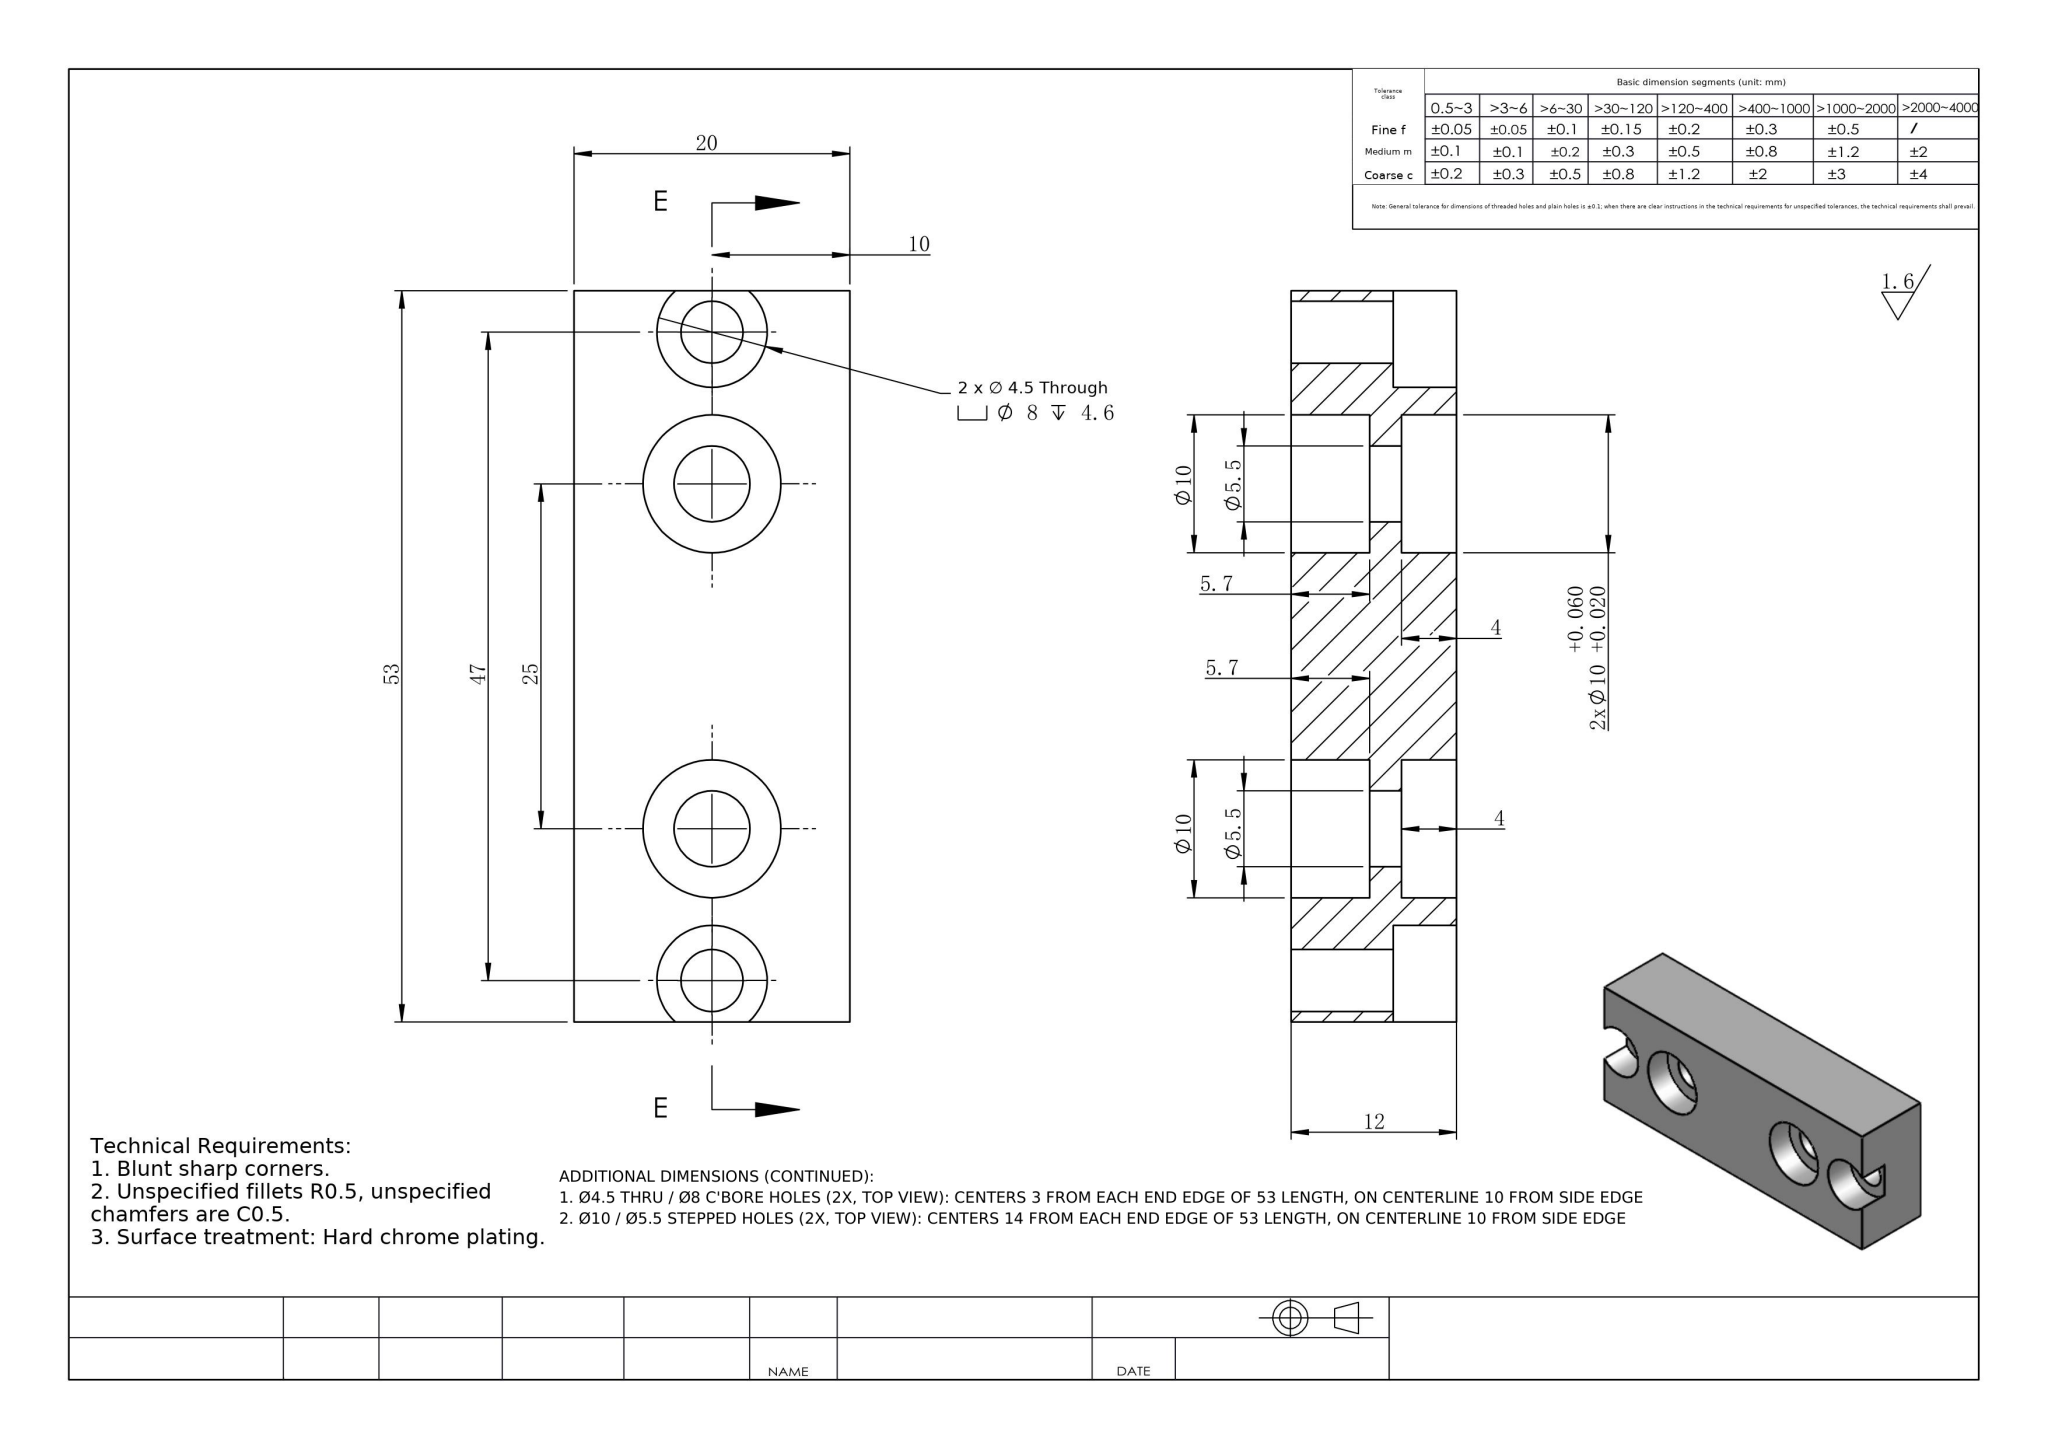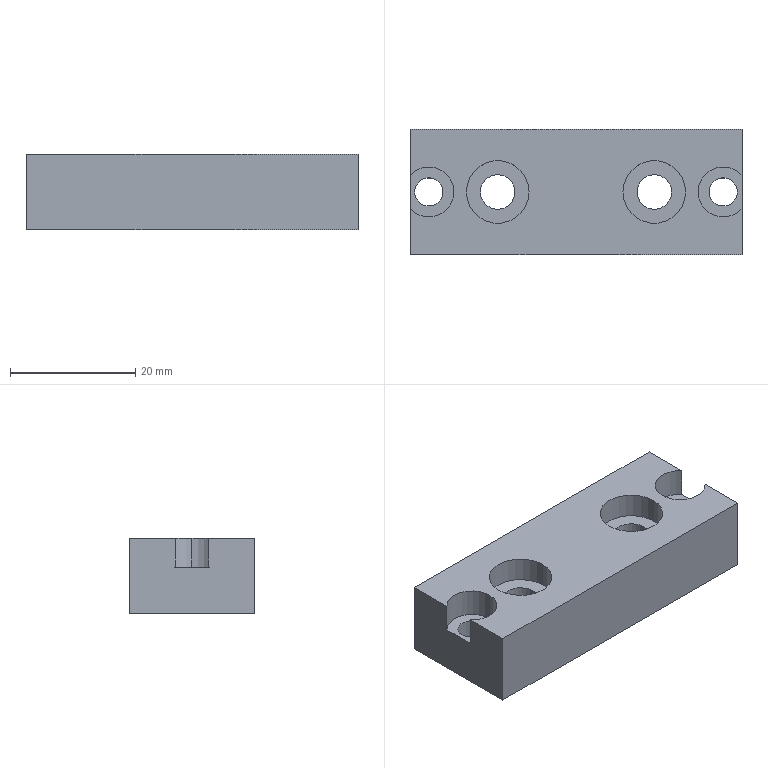Part | NX | mm | 1 solid | 31 faces | box 53 x 20 x 12 mm | volume 10423 mm3 | cylinder 19 | plane 12 | commonest cylinder face diameters 10 x8 5.5 x4 4.5 x4 8 x3
STEP:
#1=COLOUR_RGB('',1.,1.,1.);
#2=FILL_AREA_STYLE_COLOUR('',#1);
#3=FILL_AREA_STYLE('',(#2));
#4=SURFACE_STYLE_FILL_AREA(#3);
#5=SURFACE_SIDE_STYLE('',(#4));
#6=SURFACE_STYLE_USAGE(.BOTH.,#5);
#7=PRESENTATION_STYLE_ASSIGNMENT((#6));
#8=CARTESIAN_POINT('',(44.,-10.,5.7));
#9=VERTEX_POINT('',#8);
#10=CARTESIAN_POINT('',(34.,-10.,5.7));
#11=VERTEX_POINT('',#10);
#12=CARTESIAN_POINT('',(39.,-10.,5.7));
#13=DIRECTION('',(0.,0.,-1.));
#14=DIRECTION('',(-1.,0.,0.));
#15=AXIS2_PLACEMENT_3D('',#12,#13,#14);
#16=CIRCLE('',#15,5.);
#17=EDGE_CURVE('',#9,#11,#16,.T.);
#18=ORIENTED_EDGE('',*,*,#17,.F.);
#19=CARTESIAN_POINT('',(44.,-10.,0.));
#20=VERTEX_POINT('',#19);
#21=CARTESIAN_POINT('',(44.,-10.,0.));
#22=DIRECTION('',(0.,0.,-1.));
#23=VECTOR('',#22,1000.);
#24=LINE('',#21,#23);
#25=EDGE_CURVE('',#9,#20,#24,.T.);
#26=ORIENTED_EDGE('',*,*,#25,.T.);
#27=CARTESIAN_POINT('',(34.,-10.,0.));
#28=VERTEX_POINT('',#27);
#29=CARTESIAN_POINT('',(39.,-10.,0.));
#30=DIRECTION('',(0.,0.,-1.));
#31=DIRECTION('',(-1.,0.,0.));
#32=AXIS2_PLACEMENT_3D('',#29,#30,#31);
#33=CIRCLE('',#32,5.);
#34=EDGE_CURVE('',#20,#28,#33,.T.);
#35=ORIENTED_EDGE('',*,*,#34,.T.);
#36=CARTESIAN_POINT('',(34.,-10.,0.));
#37=DIRECTION('',(0.,0.,-1.));
#38=VECTOR('',#37,1000.);
#39=LINE('',#36,#38);
#40=EDGE_CURVE('',#11,#28,#39,.T.);
#41=ORIENTED_EDGE('',*,*,#40,.F.);
#42=EDGE_LOOP('',(#18,#26,#35,#41));
#43=FACE_OUTER_BOUND('',#42,.T.);
#44=CARTESIAN_POINT('',(39.,-10.,0.));
#45=DIRECTION('',(0.,0.,-1.));
#46=DIRECTION('',(-1.,0.,0.));
#47=AXIS2_PLACEMENT_3D('',#44,#45,#46);
#48=CYLINDRICAL_SURFACE('',#47,5.);
#49=ADVANCED_FACE('',(#43),#48,.F.);
#50=CARTESIAN_POINT('',(36.25,-10.,8.));
#51=VERTEX_POINT('',#50);
#52=CARTESIAN_POINT('',(41.75,-10.,8.));
#53=VERTEX_POINT('',#52);
#54=CARTESIAN_POINT('',(39.,-10.,8.));
#55=DIRECTION('',(0.,0.,1.));
#56=DIRECTION('',(1.,0.,0.));
#57=AXIS2_PLACEMENT_3D('',#54,#55,#56);
#58=CIRCLE('',#57,2.75);
#59=EDGE_CURVE('',#51,#53,#58,.T.);
#60=ORIENTED_EDGE('',*,*,#59,.T.);
#61=CARTESIAN_POINT('',(41.75,-10.,5.7));
#62=VERTEX_POINT('',#61);
#63=CARTESIAN_POINT('',(41.75,-10.,0.));
#64=DIRECTION('',(0.,0.,-1.));
#65=VECTOR('',#64,1000.);
#66=LINE('',#63,#65);
#67=EDGE_CURVE('',#53,#62,#66,.T.);
#68=ORIENTED_EDGE('',*,*,#67,.T.);
#69=CARTESIAN_POINT('',(36.25,-10.,5.7));
#70=VERTEX_POINT('',#69);
#71=CARTESIAN_POINT('',(39.,-10.,5.7));
#72=DIRECTION('',(0.,0.,-1.));
#73=DIRECTION('',(-1.,0.,0.));
#74=AXIS2_PLACEMENT_3D('',#71,#72,#73);
#75=CIRCLE('',#74,2.75);
#76=EDGE_CURVE('',#62,#70,#75,.T.);
#77=ORIENTED_EDGE('',*,*,#76,.T.);
#78=CARTESIAN_POINT('',(36.25,-10.,0.));
#79=DIRECTION('',(0.,0.,-1.));
#80=VECTOR('',#79,1000.);
#81=LINE('',#78,#80);
#82=EDGE_CURVE('',#51,#70,#81,.T.);
#83=ORIENTED_EDGE('',*,*,#82,.F.);
#84=EDGE_LOOP('',(#60,#68,#77,#83));
#85=FACE_OUTER_BOUND('',#84,.T.);
#86=CARTESIAN_POINT('',(39.,-10.,0.));
#87=DIRECTION('',(0.,0.,-1.));
#88=DIRECTION('',(-1.,0.,0.));
#89=AXIS2_PLACEMENT_3D('',#86,#87,#88);
#90=CYLINDRICAL_SURFACE('',#89,2.75);
#91=ADVANCED_FACE('',(#85),#90,.F.);
#92=CARTESIAN_POINT('',(19.,-10.,5.7));
#93=VERTEX_POINT('',#92);
#94=CARTESIAN_POINT('',(9.,-10.,5.7));
#95=VERTEX_POINT('',#94);
#96=CARTESIAN_POINT('',(14.,-10.,5.7));
#97=DIRECTION('',(0.,0.,-1.));
#98=DIRECTION('',(-1.,0.,0.));
#99=AXIS2_PLACEMENT_3D('',#96,#97,#98);
#100=CIRCLE('',#99,5.);
#101=EDGE_CURVE('',#93,#95,#100,.T.);
#102=ORIENTED_EDGE('',*,*,#101,.F.);
#103=CARTESIAN_POINT('',(19.,-10.,0.));
#104=VERTEX_POINT('',#103);
#105=CARTESIAN_POINT('',(19.,-10.,0.));
#106=DIRECTION('',(0.,0.,-1.));
#107=VECTOR('',#106,1000.);
#108=LINE('',#105,#107);
#109=EDGE_CURVE('',#93,#104,#108,.T.);
#110=ORIENTED_EDGE('',*,*,#109,.T.);
#111=CARTESIAN_POINT('',(9.,-10.,0.));
#112=VERTEX_POINT('',#111);
#113=CARTESIAN_POINT('',(14.,-10.,0.));
#114=DIRECTION('',(0.,0.,-1.));
#115=DIRECTION('',(-1.,0.,0.));
#116=AXIS2_PLACEMENT_3D('',#113,#114,#115);
#117=CIRCLE('',#116,5.);
#118=EDGE_CURVE('',#104,#112,#117,.T.);
#119=ORIENTED_EDGE('',*,*,#118,.T.);
#120=CARTESIAN_POINT('',(9.,-10.,0.));
#121=DIRECTION('',(0.,0.,-1.));
#122=VECTOR('',#121,1000.);
#123=LINE('',#120,#122);
#124=EDGE_CURVE('',#95,#112,#123,.T.);
#125=ORIENTED_EDGE('',*,*,#124,.F.);
#126=EDGE_LOOP('',(#102,#110,#119,#125));
#127=FACE_OUTER_BOUND('',#126,.T.);
#128=CARTESIAN_POINT('',(14.,-10.,0.));
#129=DIRECTION('',(0.,0.,-1.));
#130=DIRECTION('',(-1.,0.,0.));
#131=AXIS2_PLACEMENT_3D('',#128,#129,#130);
#132=CYLINDRICAL_SURFACE('',#131,5.);
#133=ADVANCED_FACE('',(#127),#132,.F.);
#134=CARTESIAN_POINT('',(11.25,-10.,8.));
#135=VERTEX_POINT('',#134);
#136=CARTESIAN_POINT('',(16.75,-10.,8.));
#137=VERTEX_POINT('',#136);
#138=CARTESIAN_POINT('',(14.,-10.,8.));
#139=DIRECTION('',(0.,0.,1.));
#140=DIRECTION('',(1.,0.,0.));
#141=AXIS2_PLACEMENT_3D('',#138,#139,#140);
#142=CIRCLE('',#141,2.75);
#143=EDGE_CURVE('',#135,#137,#142,.T.);
#144=ORIENTED_EDGE('',*,*,#143,.T.);
#145=CARTESIAN_POINT('',(16.75,-10.,5.7));
#146=VERTEX_POINT('',#145);
#147=CARTESIAN_POINT('',(16.75,-10.,0.));
#148=DIRECTION('',(0.,0.,-1.));
#149=VECTOR('',#148,1000.);
#150=LINE('',#147,#149);
#151=EDGE_CURVE('',#137,#146,#150,.T.);
#152=ORIENTED_EDGE('',*,*,#151,.T.);
#153=CARTESIAN_POINT('',(11.25,-10.,5.7));
#154=VERTEX_POINT('',#153);
#155=CARTESIAN_POINT('',(14.,-10.,5.7));
#156=DIRECTION('',(0.,0.,-1.));
#157=DIRECTION('',(-1.,0.,0.));
#158=AXIS2_PLACEMENT_3D('',#155,#156,#157);
#159=CIRCLE('',#158,2.75);
#160=EDGE_CURVE('',#146,#154,#159,.T.);
#161=ORIENTED_EDGE('',*,*,#160,.T.);
#162=CARTESIAN_POINT('',(11.25,-10.,0.));
#163=DIRECTION('',(0.,0.,-1.));
#164=VECTOR('',#163,1000.);
#165=LINE('',#162,#164);
#166=EDGE_CURVE('',#135,#154,#165,.T.);
#167=ORIENTED_EDGE('',*,*,#166,.F.);
#168=EDGE_LOOP('',(#144,#152,#161,#167));
#169=FACE_OUTER_BOUND('',#168,.T.);
#170=CARTESIAN_POINT('',(14.,-10.,0.));
#171=DIRECTION('',(0.,0.,-1.));
#172=DIRECTION('',(-1.,0.,0.));
#173=AXIS2_PLACEMENT_3D('',#170,#171,#172);
#174=CYLINDRICAL_SURFACE('',#173,2.75);
#175=ADVANCED_FACE('',(#169),#174,.F.);
#176=CARTESIAN_POINT('',(34.,-10.,8.));
#177=VERTEX_POINT('',#176);
#178=CARTESIAN_POINT('',(44.,-10.,8.));
#179=VERTEX_POINT('',#178);
#180=CARTESIAN_POINT('',(39.,-10.,8.));
#181=DIRECTION('',(0.,0.,1.));
#182=DIRECTION('',(1.,0.,0.));
#183=AXIS2_PLACEMENT_3D('',#180,#181,#182);
#184=CIRCLE('',#183,5.);
#185=EDGE_CURVE('',#177,#179,#184,.T.);
#186=ORIENTED_EDGE('',*,*,#185,.F.);
#187=CARTESIAN_POINT('',(34.,-10.,12.));
#188=VERTEX_POINT('',#187);
#189=CARTESIAN_POINT('',(34.,-10.,8.));
#190=DIRECTION('',(0.,0.,1.));
#191=VECTOR('',#190,1000.);
#192=LINE('',#189,#191);
#193=EDGE_CURVE('',#177,#188,#192,.T.);
#194=ORIENTED_EDGE('',*,*,#193,.T.);
#195=CARTESIAN_POINT('',(44.,-10.,12.));
#196=VERTEX_POINT('',#195);
#197=CARTESIAN_POINT('',(39.,-10.,12.));
#198=DIRECTION('',(0.,0.,1.));
#199=DIRECTION('',(1.,0.,0.));
#200=AXIS2_PLACEMENT_3D('',#197,#198,#199);
#201=CIRCLE('',#200,5.);
#202=EDGE_CURVE('',#188,#196,#201,.T.);
#203=ORIENTED_EDGE('',*,*,#202,.T.);
#204=CARTESIAN_POINT('',(44.,-10.,8.));
#205=DIRECTION('',(0.,0.,1.));
#206=VECTOR('',#205,1000.);
#207=LINE('',#204,#206);
#208=EDGE_CURVE('',#179,#196,#207,.T.);
#209=ORIENTED_EDGE('',*,*,#208,.F.);
#210=EDGE_LOOP('',(#186,#194,#203,#209));
#211=FACE_OUTER_BOUND('',#210,.T.);
#212=CARTESIAN_POINT('',(39.,-10.,8.));
#213=DIRECTION('',(0.,0.,1.));
#214=DIRECTION('',(1.,0.,0.));
#215=AXIS2_PLACEMENT_3D('',#212,#213,#214);
#216=CYLINDRICAL_SURFACE('',#215,5.);
#217=ADVANCED_FACE('',(#211),#216,.F.);
#218=CARTESIAN_POINT('',(9.,-10.,8.));
#219=VERTEX_POINT('',#218);
#220=CARTESIAN_POINT('',(19.,-10.,8.));
#221=VERTEX_POINT('',#220);
#222=CARTESIAN_POINT('',(14.,-10.,8.));
#223=DIRECTION('',(0.,0.,1.));
#224=DIRECTION('',(1.,0.,0.));
#225=AXIS2_PLACEMENT_3D('',#222,#223,#224);
#226=CIRCLE('',#225,5.);
#227=EDGE_CURVE('',#219,#221,#226,.T.);
#228=ORIENTED_EDGE('',*,*,#227,.F.);
#229=CARTESIAN_POINT('',(9.,-10.,12.));
#230=VERTEX_POINT('',#229);
#231=CARTESIAN_POINT('',(9.,-10.,8.));
#232=DIRECTION('',(0.,0.,1.));
#233=VECTOR('',#232,1000.);
#234=LINE('',#231,#233);
#235=EDGE_CURVE('',#219,#230,#234,.T.);
#236=ORIENTED_EDGE('',*,*,#235,.T.);
#237=CARTESIAN_POINT('',(19.,-10.,12.));
#238=VERTEX_POINT('',#237);
#239=CARTESIAN_POINT('',(14.,-10.,12.));
#240=DIRECTION('',(0.,0.,1.));
#241=DIRECTION('',(1.,0.,0.));
#242=AXIS2_PLACEMENT_3D('',#239,#240,#241);
#243=CIRCLE('',#242,5.);
#244=EDGE_CURVE('',#230,#238,#243,.T.);
#245=ORIENTED_EDGE('',*,*,#244,.T.);
#246=CARTESIAN_POINT('',(19.,-10.,8.));
#247=DIRECTION('',(0.,0.,1.));
#248=VECTOR('',#247,1000.);
#249=LINE('',#246,#248);
#250=EDGE_CURVE('',#221,#238,#249,.T.);
#251=ORIENTED_EDGE('',*,*,#250,.F.);
#252=EDGE_LOOP('',(#228,#236,#245,#251));
#253=FACE_OUTER_BOUND('',#252,.T.);
#254=CARTESIAN_POINT('',(14.,-10.,8.));
#255=DIRECTION('',(0.,0.,1.));
#256=DIRECTION('',(1.,0.,0.));
#257=AXIS2_PLACEMENT_3D('',#254,#255,#256);
#258=CYLINDRICAL_SURFACE('',#257,5.);
#259=ADVANCED_FACE('',(#253),#258,.F.);
#260=CARTESIAN_POINT('',(0.75,-10.,0.));
#261=VERTEX_POINT('',#260);
#262=CARTESIAN_POINT('',(5.25,-10.,0.));
#263=VERTEX_POINT('',#262);
#264=CARTESIAN_POINT('',(3.,-10.,0.));
#265=DIRECTION('',(0.,0.,1.));
#266=DIRECTION('',(1.,0.,0.));
#267=AXIS2_PLACEMENT_3D('',#264,#265,#266);
#268=CIRCLE('',#267,2.25);
#269=EDGE_CURVE('',#261,#263,#268,.T.);
#270=ORIENTED_EDGE('',*,*,#269,.F.);
#271=CARTESIAN_POINT('',(0.75,-10.,7.4));
#272=VERTEX_POINT('',#271);
#273=CARTESIAN_POINT('',(0.75,-10.,12.));
#274=DIRECTION('',(0.,0.,1.));
#275=VECTOR('',#274,1000.);
#276=LINE('',#273,#275);
#277=EDGE_CURVE('',#261,#272,#276,.T.);
#278=ORIENTED_EDGE('',*,*,#277,.T.);
#279=CARTESIAN_POINT('',(5.25,-10.,7.4));
#280=VERTEX_POINT('',#279);
#281=CARTESIAN_POINT('',(3.,-10.,7.4));
#282=DIRECTION('',(0.,0.,1.));
#283=DIRECTION('',(1.,0.,0.));
#284=AXIS2_PLACEMENT_3D('',#281,#282,#283);
#285=CIRCLE('',#284,2.25);
#286=EDGE_CURVE('',#272,#280,#285,.T.);
#287=ORIENTED_EDGE('',*,*,#286,.T.);
#288=CARTESIAN_POINT('',(5.25,-10.,12.));
#289=DIRECTION('',(0.,0.,1.));
#290=VECTOR('',#289,1000.);
#291=LINE('',#288,#290);
#292=EDGE_CURVE('',#263,#280,#291,.T.);
#293=ORIENTED_EDGE('',*,*,#292,.F.);
#294=EDGE_LOOP('',(#270,#278,#287,#293));
#295=FACE_OUTER_BOUND('',#294,.T.);
#296=CARTESIAN_POINT('',(3.,-10.,12.));
#297=DIRECTION('',(0.,0.,1.));
#298=DIRECTION('',(1.,0.,0.));
#299=AXIS2_PLACEMENT_3D('',#296,#297,#298);
#300=CYLINDRICAL_SURFACE('',#299,2.25);
#301=ADVANCED_FACE('',(#295),#300,.F.);
#302=CARTESIAN_POINT('',(7.,-10.,7.4));
#303=VERTEX_POINT('',#302);
#304=CARTESIAN_POINT('',(0.,-7.354,7.4));
#305=VERTEX_POINT('',#304);
#306=CARTESIAN_POINT('',(3.,-10.,7.4));
#307=DIRECTION('',(0.,0.,1.));
#308=DIRECTION('',(1.,0.,0.));
#309=AXIS2_PLACEMENT_3D('',#306,#307,#308);
#310=CIRCLE('',#309,4.);
#311=EDGE_CURVE('',#303,#305,#310,.T.);
#312=ORIENTED_EDGE('',*,*,#311,.F.);
#313=CARTESIAN_POINT('',(7.,-10.,12.));
#314=VERTEX_POINT('',#313);
#315=CARTESIAN_POINT('',(7.,-10.,12.));
#316=DIRECTION('',(0.,0.,1.));
#317=VECTOR('',#316,1000.);
#318=LINE('',#315,#317);
#319=EDGE_CURVE('',#303,#314,#318,.T.);
#320=ORIENTED_EDGE('',*,*,#319,.T.);
#321=CARTESIAN_POINT('',(0.,-7.354,12.));
#322=VERTEX_POINT('',#321);
#323=CARTESIAN_POINT('',(3.,-10.,12.));
#324=DIRECTION('',(0.,0.,1.));
#325=DIRECTION('',(1.,0.,0.));
#326=AXIS2_PLACEMENT_3D('',#323,#324,#325);
#327=CIRCLE('',#326,4.);
#328=EDGE_CURVE('',#314,#322,#327,.T.);
#329=ORIENTED_EDGE('',*,*,#328,.T.);
#330=CARTESIAN_POINT('',(0.,-7.354,12.));
#331=DIRECTION('',(0.,0.,1.));
#332=VECTOR('',#331,1000.);
#333=LINE('',#330,#332);
#334=EDGE_CURVE('',#305,#322,#333,.T.);
#335=ORIENTED_EDGE('',*,*,#334,.F.);
#336=EDGE_LOOP('',(#312,#320,#329,#335));
#337=FACE_OUTER_BOUND('',#336,.T.);
#338=CARTESIAN_POINT('',(3.,-10.,12.));
#339=DIRECTION('',(0.,0.,1.));
#340=DIRECTION('',(1.,0.,0.));
#341=AXIS2_PLACEMENT_3D('',#338,#339,#340);
#342=CYLINDRICAL_SURFACE('',#341,4.);
#343=ADVANCED_FACE('',(#337),#342,.F.);
#344=CARTESIAN_POINT('',(47.75,-10.,0.));
#345=VERTEX_POINT('',#344);
#346=CARTESIAN_POINT('',(52.25,-10.,0.));
#347=VERTEX_POINT('',#346);
#348=CARTESIAN_POINT('',(50.,-10.,0.));
#349=DIRECTION('',(0.,0.,1.));
#350=DIRECTION('',(1.,0.,0.));
#351=AXIS2_PLACEMENT_3D('',#348,#349,#350);
#352=CIRCLE('',#351,2.25);
#353=EDGE_CURVE('',#345,#347,#352,.T.);
#354=ORIENTED_EDGE('',*,*,#353,.F.);
#355=CARTESIAN_POINT('',(47.75,-10.,7.4));
#356=VERTEX_POINT('',#355);
#357=CARTESIAN_POINT('',(47.75,-10.,12.));
#358=DIRECTION('',(0.,0.,1.));
#359=VECTOR('',#358,1000.);
#360=LINE('',#357,#359);
#361=EDGE_CURVE('',#345,#356,#360,.T.);
#362=ORIENTED_EDGE('',*,*,#361,.T.);
#363=CARTESIAN_POINT('',(52.25,-10.,7.4));
#364=VERTEX_POINT('',#363);
#365=CARTESIAN_POINT('',(50.,-10.,7.4));
#366=DIRECTION('',(0.,0.,1.));
#367=DIRECTION('',(1.,0.,0.));
#368=AXIS2_PLACEMENT_3D('',#365,#366,#367);
#369=CIRCLE('',#368,2.25);
#370=EDGE_CURVE('',#356,#364,#369,.T.);
#371=ORIENTED_EDGE('',*,*,#370,.T.);
#372=CARTESIAN_POINT('',(52.25,-10.,12.));
#373=DIRECTION('',(0.,0.,1.));
#374=VECTOR('',#373,1000.);
#375=LINE('',#372,#374);
#376=EDGE_CURVE('',#347,#364,#375,.T.);
#377=ORIENTED_EDGE('',*,*,#376,.F.);
#378=EDGE_LOOP('',(#354,#362,#371,#377));
#379=FACE_OUTER_BOUND('',#378,.T.);
#380=CARTESIAN_POINT('',(50.,-10.,12.));
#381=DIRECTION('',(0.,0.,1.));
#382=DIRECTION('',(1.,0.,0.));
#383=AXIS2_PLACEMENT_3D('',#380,#381,#382);
#384=CYLINDRICAL_SURFACE('',#383,2.25);
#385=ADVANCED_FACE('',(#379),#384,.F.);
#386=CARTESIAN_POINT('',(53.,0.,0.));
#387=VERTEX_POINT('',#386);
#388=CARTESIAN_POINT('',(0.,0.,0.));
#389=VERTEX_POINT('',#388);
#390=CARTESIAN_POINT('',(53.,0.,0.));
#391=DIRECTION('',(-1.,-0.,0.));
#392=VECTOR('',#391,1000.);
#393=LINE('',#390,#392);
#394=EDGE_CURVE('',#387,#389,#393,.T.);
#395=ORIENTED_EDGE('',*,*,#394,.T.);
#396=CARTESIAN_POINT('',(0.,0.,12.));
#397=VERTEX_POINT('',#396);
#398=CARTESIAN_POINT('',(0.,0.,12.));
#399=DIRECTION('',(0.,0.,-1.));
#400=VECTOR('',#399,1000.);
#401=LINE('',#398,#400);
#402=EDGE_CURVE('',#397,#389,#401,.T.);
#403=ORIENTED_EDGE('',*,*,#402,.F.);
#404=CARTESIAN_POINT('',(53.,0.,12.));
#405=VERTEX_POINT('',#404);
#406=CARTESIAN_POINT('',(53.,0.,12.));
#407=DIRECTION('',(-1.,-0.,0.));
#408=VECTOR('',#407,1000.);
#409=LINE('',#406,#408);
#410=EDGE_CURVE('',#405,#397,#409,.T.);
#411=ORIENTED_EDGE('',*,*,#410,.F.);
#412=CARTESIAN_POINT('',(53.,0.,12.));
#413=DIRECTION('',(0.,0.,-1.));
#414=VECTOR('',#413,1000.);
#415=LINE('',#412,#414);
#416=EDGE_CURVE('',#405,#387,#415,.T.);
#417=ORIENTED_EDGE('',*,*,#416,.T.);
#418=EDGE_LOOP('',(#395,#403,#411,#417));
#419=FACE_OUTER_BOUND('',#418,.T.);
#420=CARTESIAN_POINT('',(53.,0.,12.));
#421=DIRECTION('',(0.,-1.,0.));
#422=DIRECTION('',(1.,0.,0.));
#423=AXIS2_PLACEMENT_3D('',#420,#421,#422);
#424=PLANE('',#423);
#425=ADVANCED_FACE('',(#419),#424,.F.);
#426=CARTESIAN_POINT('',(0.,-12.646,7.4));
#427=VERTEX_POINT('',#426);
#428=CARTESIAN_POINT('',(0.,0.,7.4));
#429=DIRECTION('',(-0.,1.,0.));
#430=VECTOR('',#429,1000.);
#431=LINE('',#428,#430);
#432=EDGE_CURVE('',#427,#305,#431,.T.);
#433=ORIENTED_EDGE('',*,*,#432,.T.);
#434=ORIENTED_EDGE('',*,*,#334,.T.);
#435=CARTESIAN_POINT('',(0.,0.,12.));
#436=DIRECTION('',(0.,-1.,0.));
#437=VECTOR('',#436,1000.);
#438=LINE('',#435,#437);
#439=EDGE_CURVE('',#397,#322,#438,.T.);
#440=ORIENTED_EDGE('',*,*,#439,.F.);
#441=ORIENTED_EDGE('',*,*,#402,.T.);
#442=CARTESIAN_POINT('',(0.,-20.,0.));
#443=VERTEX_POINT('',#442);
#444=CARTESIAN_POINT('',(0.,0.,0.));
#445=DIRECTION('',(0.,-1.,0.));
#446=VECTOR('',#445,1000.);
#447=LINE('',#444,#446);
#448=EDGE_CURVE('',#389,#443,#447,.T.);
#449=ORIENTED_EDGE('',*,*,#448,.T.);
#450=CARTESIAN_POINT('',(0.,-20.,12.));
#451=VERTEX_POINT('',#450);
#452=CARTESIAN_POINT('',(0.,-20.,12.));
#453=DIRECTION('',(0.,0.,-1.));
#454=VECTOR('',#453,1000.);
#455=LINE('',#452,#454);
#456=EDGE_CURVE('',#451,#443,#455,.T.);
#457=ORIENTED_EDGE('',*,*,#456,.F.);
#458=CARTESIAN_POINT('',(0.,-12.646,12.));
#459=VERTEX_POINT('',#458);
#460=CARTESIAN_POINT('',(0.,0.,12.));
#461=DIRECTION('',(0.,-1.,0.));
#462=VECTOR('',#461,1000.);
#463=LINE('',#460,#462);
#464=EDGE_CURVE('',#459,#451,#463,.T.);
#465=ORIENTED_EDGE('',*,*,#464,.F.);
#466=CARTESIAN_POINT('',(0.,-12.646,12.));
#467=DIRECTION('',(0.,0.,-1.));
#468=VECTOR('',#467,1000.);
#469=LINE('',#466,#468);
#470=EDGE_CURVE('',#459,#427,#469,.T.);
#471=ORIENTED_EDGE('',*,*,#470,.T.);
#472=EDGE_LOOP('',(#433,#434,#440,#441,#449,#457,#465,#471));
#473=FACE_OUTER_BOUND('',#472,.T.);
#474=CARTESIAN_POINT('',(0.,0.,12.));
#475=DIRECTION('',(1.,0.,0.));
#476=DIRECTION('',(-0.,1.,0.));
#477=AXIS2_PLACEMENT_3D('',#474,#475,#476);
#478=PLANE('',#477);
#479=ADVANCED_FACE('',(#473),#478,.F.);
#480=CARTESIAN_POINT('',(53.,-20.,0.));
#481=VERTEX_POINT('',#480);
#482=CARTESIAN_POINT('',(0.,-20.,0.));
#483=DIRECTION('',(1.,0.,0.));
#484=VECTOR('',#483,1000.);
#485=LINE('',#482,#484);
#486=EDGE_CURVE('',#443,#481,#485,.T.);
#487=ORIENTED_EDGE('',*,*,#486,.T.);
#488=CARTESIAN_POINT('',(53.,-20.,12.));
#489=VERTEX_POINT('',#488);
#490=CARTESIAN_POINT('',(53.,-20.,12.));
#491=DIRECTION('',(0.,0.,-1.));
#492=VECTOR('',#491,1000.);
#493=LINE('',#490,#492);
#494=EDGE_CURVE('',#489,#481,#493,.T.);
#495=ORIENTED_EDGE('',*,*,#494,.F.);
#496=CARTESIAN_POINT('',(0.,-20.,12.));
#497=DIRECTION('',(1.,0.,0.));
#498=VECTOR('',#497,1000.);
#499=LINE('',#496,#498);
#500=EDGE_CURVE('',#451,#489,#499,.T.);
#501=ORIENTED_EDGE('',*,*,#500,.F.);
#502=ORIENTED_EDGE('',*,*,#456,.T.);
#503=EDGE_LOOP('',(#487,#495,#501,#502));
#504=FACE_OUTER_BOUND('',#503,.T.);
#505=CARTESIAN_POINT('',(0.,-20.,12.));
#506=DIRECTION('',(0.,1.,0.));
#507=DIRECTION('',(0.,0.,1.));
#508=AXIS2_PLACEMENT_3D('',#505,#506,#507);
#509=PLANE('',#508);
#510=ADVANCED_FACE('',(#504),#509,.F.);
#511=CARTESIAN_POINT('',(53.,-7.354,7.4));
#512=VERTEX_POINT('',#511);
#513=CARTESIAN_POINT('',(53.,-12.646,7.4));
#514=VERTEX_POINT('',#513);
#515=CARTESIAN_POINT('',(53.,-20.,7.4));
#516=DIRECTION('',(0.,-1.,0.));
#517=VECTOR('',#516,1000.);
#518=LINE('',#515,#517);
#519=EDGE_CURVE('',#512,#514,#518,.T.);
#520=ORIENTED_EDGE('',*,*,#519,.T.);
#521=CARTESIAN_POINT('',(53.,-12.646,12.));
#522=VERTEX_POINT('',#521);
#523=CARTESIAN_POINT('',(53.,-12.646,12.));
#524=DIRECTION('',(0.,0.,1.));
#525=VECTOR('',#524,1000.);
#526=LINE('',#523,#525);
#527=EDGE_CURVE('',#514,#522,#526,.T.);
#528=ORIENTED_EDGE('',*,*,#527,.T.);
#529=CARTESIAN_POINT('',(53.,-20.,12.));
#530=DIRECTION('',(0.,1.,0.));
#531=VECTOR('',#530,1000.);
#532=LINE('',#529,#531);
#533=EDGE_CURVE('',#489,#522,#532,.T.);
#534=ORIENTED_EDGE('',*,*,#533,.F.);
#535=ORIENTED_EDGE('',*,*,#494,.T.);
#536=CARTESIAN_POINT('',(53.,-20.,0.));
#537=DIRECTION('',(0.,1.,0.));
#538=VECTOR('',#537,1000.);
#539=LINE('',#536,#538);
#540=EDGE_CURVE('',#481,#387,#539,.T.);
#541=ORIENTED_EDGE('',*,*,#540,.T.);
#542=ORIENTED_EDGE('',*,*,#416,.F.);
#543=CARTESIAN_POINT('',(53.,-7.354,12.));
#544=VERTEX_POINT('',#543);
#545=CARTESIAN_POINT('',(53.,-20.,12.));
#546=DIRECTION('',(0.,1.,0.));
#547=VECTOR('',#546,1000.);
#548=LINE('',#545,#547);
#549=EDGE_CURVE('',#544,#405,#548,.T.);
#550=ORIENTED_EDGE('',*,*,#549,.F.);
#551=CARTESIAN_POINT('',(53.,-7.354,12.));
#552=DIRECTION('',(0.,0.,-1.));
#553=VECTOR('',#552,1000.);
#554=LINE('',#551,#553);
#555=EDGE_CURVE('',#544,#512,#554,.T.);
#556=ORIENTED_EDGE('',*,*,#555,.T.);
#557=EDGE_LOOP('',(#520,#528,#534,#535,#541,#542,#550,#556));
#558=FACE_OUTER_BOUND('',#557,.T.);
#559=CARTESIAN_POINT('',(53.,-20.,12.));
#560=DIRECTION('',(-1.,0.,0.));
#561=DIRECTION('',(0.,0.,1.));
#562=AXIS2_PLACEMENT_3D('',#559,#560,#561);
#563=PLANE('',#562);
#564=ADVANCED_FACE('',(#558),#563,.F.);
#565=CARTESIAN_POINT('',(39.,-10.,12.));
#566=DIRECTION('',(0.,0.,1.));
#567=DIRECTION('',(1.,0.,0.));
#568=AXIS2_PLACEMENT_3D('',#565,#566,#567);
#569=CIRCLE('',#568,5.);
#570=EDGE_CURVE('',#196,#188,#569,.T.);
#571=ORIENTED_EDGE('',*,*,#570,.F.);
#572=ORIENTED_EDGE('',*,*,#202,.F.);
#573=EDGE_LOOP('',(#571,#572));
#574=FACE_BOUND('',#573,.T.);
#575=CARTESIAN_POINT('',(14.,-10.,12.));
#576=DIRECTION('',(0.,0.,1.));
#577=DIRECTION('',(1.,0.,0.));
#578=AXIS2_PLACEMENT_3D('',#575,#576,#577);
#579=CIRCLE('',#578,5.);
#580=EDGE_CURVE('',#238,#230,#579,.T.);
#581=ORIENTED_EDGE('',*,*,#580,.F.);
#582=ORIENTED_EDGE('',*,*,#244,.F.);
#583=EDGE_LOOP('',(#581,#582));
#584=FACE_BOUND('',#583,.T.);
#585=CARTESIAN_POINT('',(3.,-10.,12.));
#586=DIRECTION('',(0.,0.,1.));
#587=DIRECTION('',(1.,0.,0.));
#588=AXIS2_PLACEMENT_3D('',#585,#586,#587);
#589=CIRCLE('',#588,4.);
#590=EDGE_CURVE('',#459,#314,#589,.T.);
#591=ORIENTED_EDGE('',*,*,#590,.F.);
#592=ORIENTED_EDGE('',*,*,#464,.T.);
#593=ORIENTED_EDGE('',*,*,#500,.T.);
#594=ORIENTED_EDGE('',*,*,#533,.T.);
#595=CARTESIAN_POINT('',(50.,-10.,12.));
#596=DIRECTION('',(0.,0.,1.));
#597=DIRECTION('',(1.,0.,0.));
#598=AXIS2_PLACEMENT_3D('',#595,#596,#597);
#599=CIRCLE('',#598,4.);
#600=EDGE_CURVE('',#544,#522,#599,.T.);
#601=ORIENTED_EDGE('',*,*,#600,.F.);
#602=ORIENTED_EDGE('',*,*,#549,.T.);
#603=ORIENTED_EDGE('',*,*,#410,.T.);
#604=ORIENTED_EDGE('',*,*,#439,.T.);
#605=ORIENTED_EDGE('',*,*,#328,.F.);
#606=EDGE_LOOP('',(#591,#592,#593,#594,#601,#602,#603,#604,#605));
#607=FACE_OUTER_BOUND('',#606,.T.);
#608=CARTESIAN_POINT('',(0.,0.,12.));
#609=DIRECTION('',(0.,0.,1.));
#610=DIRECTION('',(1.,0.,0.));
#611=AXIS2_PLACEMENT_3D('',#608,#609,#610);
#612=PLANE('',#611);
#613=ADVANCED_FACE('',(#574,#584,#607),#612,.T.);
#614=CARTESIAN_POINT('',(39.,-10.,0.));
#615=DIRECTION('',(0.,0.,-1.));
#616=DIRECTION('',(-1.,0.,0.));
#617=AXIS2_PLACEMENT_3D('',#614,#615,#616);
#618=CIRCLE('',#617,5.);
#619=EDGE_CURVE('',#28,#20,#618,.T.);
#620=ORIENTED_EDGE('',*,*,#619,.F.);
#621=ORIENTED_EDGE('',*,*,#34,.F.);
#622=EDGE_LOOP('',(#620,#621));
#623=FACE_BOUND('',#622,.T.);
#624=CARTESIAN_POINT('',(14.,-10.,0.));
#625=DIRECTION('',(0.,0.,-1.));
#626=DIRECTION('',(-1.,0.,0.));
#627=AXIS2_PLACEMENT_3D('',#624,#625,#626);
#628=CIRCLE('',#627,5.);
#629=EDGE_CURVE('',#112,#104,#628,.T.);
#630=ORIENTED_EDGE('',*,*,#629,.F.);
#631=ORIENTED_EDGE('',*,*,#118,.F.);
#632=EDGE_LOOP('',(#630,#631));
#633=FACE_BOUND('',#632,.T.);
#634=CARTESIAN_POINT('',(3.,-10.,0.));
#635=DIRECTION('',(0.,0.,1.));
#636=DIRECTION('',(1.,0.,0.));
#637=AXIS2_PLACEMENT_3D('',#634,#635,#636);
#638=CIRCLE('',#637,2.25);
#639=EDGE_CURVE('',#263,#261,#638,.T.);
#640=ORIENTED_EDGE('',*,*,#639,.T.);
#641=ORIENTED_EDGE('',*,*,#269,.T.);
#642=EDGE_LOOP('',(#640,#641));
#643=FACE_BOUND('',#642,.T.);
#644=CARTESIAN_POINT('',(50.,-10.,0.));
#645=DIRECTION('',(0.,0.,1.));
#646=DIRECTION('',(1.,0.,0.));
#647=AXIS2_PLACEMENT_3D('',#644,#645,#646);
#648=CIRCLE('',#647,2.25);
#649=EDGE_CURVE('',#347,#345,#648,.T.);
#650=ORIENTED_EDGE('',*,*,#649,.T.);
#651=ORIENTED_EDGE('',*,*,#353,.T.);
#652=EDGE_LOOP('',(#650,#651));
#653=FACE_BOUND('',#652,.T.);
#654=ORIENTED_EDGE('',*,*,#394,.F.);
#655=ORIENTED_EDGE('',*,*,#540,.F.);
#656=ORIENTED_EDGE('',*,*,#486,.F.);
#657=ORIENTED_EDGE('',*,*,#448,.F.);
#658=EDGE_LOOP('',(#654,#655,#656,#657));
#659=FACE_OUTER_BOUND('',#658,.T.);
#660=CARTESIAN_POINT('',(0.,0.,0.));
#661=DIRECTION('',(0.,0.,1.));
#662=DIRECTION('',(1.,0.,0.));
#663=AXIS2_PLACEMENT_3D('',#660,#661,#662);
#664=PLANE('',#663);
#665=ADVANCED_FACE('',(#623,#633,#643,#653,#659),#664,.F.);
#666=CARTESIAN_POINT('',(50.,-10.,7.4));
#667=DIRECTION('',(0.,0.,1.));
#668=DIRECTION('',(1.,0.,0.));
#669=AXIS2_PLACEMENT_3D('',#666,#667,#668);
#670=CIRCLE('',#669,2.25);
#671=EDGE_CURVE('',#364,#356,#670,.T.);
#672=ORIENTED_EDGE('',*,*,#671,.F.);
#673=ORIENTED_EDGE('',*,*,#370,.F.);
#674=EDGE_LOOP('',(#672,#673));
#675=FACE_BOUND('',#674,.T.);
#676=CARTESIAN_POINT('',(50.,-10.,7.4));
#677=DIRECTION('',(0.,0.,1.));
#678=DIRECTION('',(1.,0.,0.));
#679=AXIS2_PLACEMENT_3D('',#676,#677,#678);
#680=CIRCLE('',#679,4.);
#681=EDGE_CURVE('',#512,#514,#680,.T.);
#682=ORIENTED_EDGE('',*,*,#681,.T.);
#683=ORIENTED_EDGE('',*,*,#519,.F.);
#684=EDGE_LOOP('',(#682,#683));
#685=FACE_OUTER_BOUND('',#684,.T.);
#686=CARTESIAN_POINT('',(52.25,-10.,7.4));
#687=DIRECTION('',(0.,0.,-1.));
#688=DIRECTION('',(-1.,0.,0.));
#689=AXIS2_PLACEMENT_3D('',#686,#687,#688);
#690=PLANE('',#689);
#691=ADVANCED_FACE('',(#675,#685),#690,.F.);
#692=ORIENTED_EDGE('',*,*,#681,.F.);
#693=ORIENTED_EDGE('',*,*,#555,.F.);
#694=ORIENTED_EDGE('',*,*,#600,.T.);
#695=ORIENTED_EDGE('',*,*,#527,.F.);
#696=EDGE_LOOP('',(#692,#693,#694,#695));
#697=FACE_OUTER_BOUND('',#696,.T.);
#698=CARTESIAN_POINT('',(50.,-10.,12.));
#699=DIRECTION('',(0.,0.,1.));
#700=DIRECTION('',(1.,0.,0.));
#701=AXIS2_PLACEMENT_3D('',#698,#699,#700);
#702=CYLINDRICAL_SURFACE('',#701,4.);
#703=ADVANCED_FACE('',(#697),#702,.F.);
#704=ORIENTED_EDGE('',*,*,#361,.F.);
#705=ORIENTED_EDGE('',*,*,#649,.F.);
#706=ORIENTED_EDGE('',*,*,#376,.T.);
#707=ORIENTED_EDGE('',*,*,#671,.T.);
#708=EDGE_LOOP('',(#704,#705,#706,#707));
#709=FACE_OUTER_BOUND('',#708,.T.);
#710=CARTESIAN_POINT('',(50.,-10.,12.));
#711=DIRECTION('',(0.,0.,1.));
#712=DIRECTION('',(1.,0.,0.));
#713=AXIS2_PLACEMENT_3D('',#710,#711,#712);
#714=CYLINDRICAL_SURFACE('',#713,2.25);
#715=ADVANCED_FACE('',(#709),#714,.F.);
#716=CARTESIAN_POINT('',(3.,-10.,7.4));
#717=DIRECTION('',(0.,0.,1.));
#718=DIRECTION('',(1.,0.,0.));
#719=AXIS2_PLACEMENT_3D('',#716,#717,#718);
#720=CIRCLE('',#719,2.25);
#721=EDGE_CURVE('',#280,#272,#720,.T.);
#722=ORIENTED_EDGE('',*,*,#721,.F.);
#723=ORIENTED_EDGE('',*,*,#286,.F.);
#724=EDGE_LOOP('',(#722,#723));
#725=FACE_BOUND('',#724,.T.);
#726=CARTESIAN_POINT('',(3.,-10.,7.4));
#727=DIRECTION('',(0.,0.,1.));
#728=DIRECTION('',(1.,0.,0.));
#729=AXIS2_PLACEMENT_3D('',#726,#727,#728);
#730=CIRCLE('',#729,4.);
#731=EDGE_CURVE('',#427,#303,#730,.T.);
#732=ORIENTED_EDGE('',*,*,#731,.T.);
#733=ORIENTED_EDGE('',*,*,#311,.T.);
#734=ORIENTED_EDGE('',*,*,#432,.F.);
#735=EDGE_LOOP('',(#732,#733,#734));
#736=FACE_OUTER_BOUND('',#735,.T.);
#737=CARTESIAN_POINT('',(5.25,-10.,7.4));
#738=DIRECTION('',(0.,0.,-1.));
#739=DIRECTION('',(-1.,0.,0.));
#740=AXIS2_PLACEMENT_3D('',#737,#738,#739);
#741=PLANE('',#740);
#742=ADVANCED_FACE('',(#725,#736),#741,.F.);
#743=ORIENTED_EDGE('',*,*,#319,.F.);
#744=ORIENTED_EDGE('',*,*,#731,.F.);
#745=ORIENTED_EDGE('',*,*,#470,.F.);
#746=ORIENTED_EDGE('',*,*,#590,.T.);
#747=EDGE_LOOP('',(#743,#744,#745,#746));
#748=FACE_OUTER_BOUND('',#747,.T.);
#749=CARTESIAN_POINT('',(3.,-10.,12.));
#750=DIRECTION('',(0.,0.,1.));
#751=DIRECTION('',(1.,0.,0.));
#752=AXIS2_PLACEMENT_3D('',#749,#750,#751);
#753=CYLINDRICAL_SURFACE('',#752,4.);
#754=ADVANCED_FACE('',(#748),#753,.F.);
#755=ORIENTED_EDGE('',*,*,#277,.F.);
#756=ORIENTED_EDGE('',*,*,#639,.F.);
#757=ORIENTED_EDGE('',*,*,#292,.T.);
#758=ORIENTED_EDGE('',*,*,#721,.T.);
#759=EDGE_LOOP('',(#755,#756,#757,#758));
#760=FACE_OUTER_BOUND('',#759,.T.);
#761=CARTESIAN_POINT('',(3.,-10.,12.));
#762=DIRECTION('',(0.,0.,1.));
#763=DIRECTION('',(1.,0.,0.));
#764=AXIS2_PLACEMENT_3D('',#761,#762,#763);
#765=CYLINDRICAL_SURFACE('',#764,2.25);
#766=ADVANCED_FACE('',(#760),#765,.F.);
#767=ORIENTED_EDGE('',*,*,#235,.F.);
#768=CARTESIAN_POINT('',(14.,-10.,8.));
#769=DIRECTION('',(0.,0.,1.));
#770=DIRECTION('',(1.,0.,0.));
#771=AXIS2_PLACEMENT_3D('',#768,#769,#770);
#772=CIRCLE('',#771,5.);
#773=EDGE_CURVE('',#221,#219,#772,.T.);
#774=ORIENTED_EDGE('',*,*,#773,.F.);
#775=ORIENTED_EDGE('',*,*,#250,.T.);
#776=ORIENTED_EDGE('',*,*,#580,.T.);
#777=EDGE_LOOP('',(#767,#774,#775,#776));
#778=FACE_OUTER_BOUND('',#777,.T.);
#779=CARTESIAN_POINT('',(14.,-10.,8.));
#780=DIRECTION('',(0.,0.,1.));
#781=DIRECTION('',(1.,0.,0.));
#782=AXIS2_PLACEMENT_3D('',#779,#780,#781);
#783=CYLINDRICAL_SURFACE('',#782,5.);
#784=ADVANCED_FACE('',(#778),#783,.F.);
#785=ORIENTED_EDGE('',*,*,#143,.F.);
#786=CARTESIAN_POINT('',(14.,-10.,8.));
#787=DIRECTION('',(0.,0.,1.));
#788=DIRECTION('',(1.,0.,0.));
#789=AXIS2_PLACEMENT_3D('',#786,#787,#788);
#790=CIRCLE('',#789,2.75);
#791=EDGE_CURVE('',#137,#135,#790,.T.);
#792=ORIENTED_EDGE('',*,*,#791,.F.);
#793=EDGE_LOOP('',(#785,#792));
#794=FACE_BOUND('',#793,.T.);
#795=ORIENTED_EDGE('',*,*,#773,.T.);
#796=ORIENTED_EDGE('',*,*,#227,.T.);
#797=EDGE_LOOP('',(#795,#796));
#798=FACE_OUTER_BOUND('',#797,.T.);
#799=CARTESIAN_POINT('',(14.,-10.,8.));
#800=DIRECTION('',(0.,0.,1.));
#801=DIRECTION('',(1.,0.,0.));
#802=AXIS2_PLACEMENT_3D('',#799,#800,#801);
#803=PLANE('',#802);
#804=ADVANCED_FACE('',(#794,#798),#803,.T.);
#805=ORIENTED_EDGE('',*,*,#193,.F.);
#806=CARTESIAN_POINT('',(39.,-10.,8.));
#807=DIRECTION('',(0.,0.,1.));
#808=DIRECTION('',(1.,0.,0.));
#809=AXIS2_PLACEMENT_3D('',#806,#807,#808);
#810=CIRCLE('',#809,5.);
#811=EDGE_CURVE('',#179,#177,#810,.T.);
#812=ORIENTED_EDGE('',*,*,#811,.F.);
#813=ORIENTED_EDGE('',*,*,#208,.T.);
#814=ORIENTED_EDGE('',*,*,#570,.T.);
#815=EDGE_LOOP('',(#805,#812,#813,#814));
#816=FACE_OUTER_BOUND('',#815,.T.);
#817=CARTESIAN_POINT('',(39.,-10.,8.));
#818=DIRECTION('',(0.,0.,1.));
#819=DIRECTION('',(1.,0.,0.));
#820=AXIS2_PLACEMENT_3D('',#817,#818,#819);
#821=CYLINDRICAL_SURFACE('',#820,5.);
#822=ADVANCED_FACE('',(#816),#821,.F.);
#823=ORIENTED_EDGE('',*,*,#59,.F.);
#824=CARTESIAN_POINT('',(39.,-10.,8.));
#825=DIRECTION('',(0.,0.,1.));
#826=DIRECTION('',(1.,0.,0.));
#827=AXIS2_PLACEMENT_3D('',#824,#825,#826);
#828=CIRCLE('',#827,2.75);
#829=EDGE_CURVE('',#53,#51,#828,.T.);
#830=ORIENTED_EDGE('',*,*,#829,.F.);
#831=EDGE_LOOP('',(#823,#830));
#832=FACE_BOUND('',#831,.T.);
#833=ORIENTED_EDGE('',*,*,#811,.T.);
#834=ORIENTED_EDGE('',*,*,#185,.T.);
#835=EDGE_LOOP('',(#833,#834));
#836=FACE_OUTER_BOUND('',#835,.T.);
#837=CARTESIAN_POINT('',(39.,-10.,8.));
#838=DIRECTION('',(0.,0.,1.));
#839=DIRECTION('',(1.,0.,0.));
#840=AXIS2_PLACEMENT_3D('',#837,#838,#839);
#841=PLANE('',#840);
#842=ADVANCED_FACE('',(#832,#836),#841,.T.);
#843=ORIENTED_EDGE('',*,*,#151,.F.);
#844=ORIENTED_EDGE('',*,*,#791,.T.);
#845=ORIENTED_EDGE('',*,*,#166,.T.);
#846=CARTESIAN_POINT('',(14.,-10.,5.7));
#847=DIRECTION('',(0.,0.,-1.));
#848=DIRECTION('',(-1.,0.,0.));
#849=AXIS2_PLACEMENT_3D('',#846,#847,#848);
#850=CIRCLE('',#849,2.75);
#851=EDGE_CURVE('',#154,#146,#850,.T.);
#852=ORIENTED_EDGE('',*,*,#851,.T.);
#853=EDGE_LOOP('',(#843,#844,#845,#852));
#854=FACE_OUTER_BOUND('',#853,.T.);
#855=CARTESIAN_POINT('',(14.,-10.,0.));
#856=DIRECTION('',(0.,0.,-1.));
#857=DIRECTION('',(-1.,0.,0.));
#858=AXIS2_PLACEMENT_3D('',#855,#856,#857);
#859=CYLINDRICAL_SURFACE('',#858,2.75);
#860=ADVANCED_FACE('',(#854),#859,.F.);
#861=ORIENTED_EDGE('',*,*,#851,.F.);
#862=ORIENTED_EDGE('',*,*,#160,.F.);
#863=EDGE_LOOP('',(#861,#862));
#864=FACE_BOUND('',#863,.T.);
#865=CARTESIAN_POINT('',(14.,-10.,5.7));
#866=DIRECTION('',(0.,0.,-1.));
#867=DIRECTION('',(-1.,0.,0.));
#868=AXIS2_PLACEMENT_3D('',#865,#866,#867);
#869=CIRCLE('',#868,5.);
#870=EDGE_CURVE('',#95,#93,#869,.T.);
#871=ORIENTED_EDGE('',*,*,#870,.T.);
#872=ORIENTED_EDGE('',*,*,#101,.T.);
#873=EDGE_LOOP('',(#871,#872));
#874=FACE_OUTER_BOUND('',#873,.T.);
#875=CARTESIAN_POINT('',(16.75,-10.,5.7));
#876=DIRECTION('',(0.,0.,1.));
#877=DIRECTION('',(1.,0.,0.));
#878=AXIS2_PLACEMENT_3D('',#875,#876,#877);
#879=PLANE('',#878);
#880=ADVANCED_FACE('',(#864,#874),#879,.F.);
#881=ORIENTED_EDGE('',*,*,#109,.F.);
#882=ORIENTED_EDGE('',*,*,#870,.F.);
#883=ORIENTED_EDGE('',*,*,#124,.T.);
#884=ORIENTED_EDGE('',*,*,#629,.T.);
#885=EDGE_LOOP('',(#881,#882,#883,#884));
#886=FACE_OUTER_BOUND('',#885,.T.);
#887=CARTESIAN_POINT('',(14.,-10.,0.));
#888=DIRECTION('',(0.,0.,-1.));
#889=DIRECTION('',(-1.,0.,0.));
#890=AXIS2_PLACEMENT_3D('',#887,#888,#889);
#891=CYLINDRICAL_SURFACE('',#890,5.);
#892=ADVANCED_FACE('',(#886),#891,.F.);
#893=ORIENTED_EDGE('',*,*,#67,.F.);
#894=ORIENTED_EDGE('',*,*,#829,.T.);
#895=ORIENTED_EDGE('',*,*,#82,.T.);
#896=CARTESIAN_POINT('',(39.,-10.,5.7));
#897=DIRECTION('',(0.,0.,-1.));
#898=DIRECTION('',(-1.,0.,0.));
#899=AXIS2_PLACEMENT_3D('',#896,#897,#898);
#900=CIRCLE('',#899,2.75);
#901=EDGE_CURVE('',#70,#62,#900,.T.);
#902=ORIENTED_EDGE('',*,*,#901,.T.);
#903=EDGE_LOOP('',(#893,#894,#895,#902));
#904=FACE_OUTER_BOUND('',#903,.T.);
#905=CARTESIAN_POINT('',(39.,-10.,0.));
#906=DIRECTION('',(0.,0.,-1.));
#907=DIRECTION('',(-1.,0.,0.));
#908=AXIS2_PLACEMENT_3D('',#905,#906,#907);
#909=CYLINDRICAL_SURFACE('',#908,2.75);
#910=ADVANCED_FACE('',(#904),#909,.F.);
#911=ORIENTED_EDGE('',*,*,#901,.F.);
#912=ORIENTED_EDGE('',*,*,#76,.F.);
#913=EDGE_LOOP('',(#911,#912));
#914=FACE_BOUND('',#913,.T.);
#915=CARTESIAN_POINT('',(39.,-10.,5.7));
#916=DIRECTION('',(0.,0.,-1.));
#917=DIRECTION('',(-1.,0.,0.));
#918=AXIS2_PLACEMENT_3D('',#915,#916,#917);
#919=CIRCLE('',#918,5.);
#920=EDGE_CURVE('',#11,#9,#919,.T.);
#921=ORIENTED_EDGE('',*,*,#920,.T.);
#922=ORIENTED_EDGE('',*,*,#17,.T.);
#923=EDGE_LOOP('',(#921,#922));
#924=FACE_OUTER_BOUND('',#923,.T.);
#925=CARTESIAN_POINT('',(41.75,-10.,5.7));
#926=DIRECTION('',(0.,0.,1.));
#927=DIRECTION('',(1.,0.,0.));
#928=AXIS2_PLACEMENT_3D('',#925,#926,#927);
#929=PLANE('',#928);
#930=ADVANCED_FACE('',(#914,#924),#929,.F.);
#931=ORIENTED_EDGE('',*,*,#25,.F.);
#932=ORIENTED_EDGE('',*,*,#920,.F.);
#933=ORIENTED_EDGE('',*,*,#40,.T.);
#934=ORIENTED_EDGE('',*,*,#619,.T.);
#935=EDGE_LOOP('',(#931,#932,#933,#934));
#936=FACE_OUTER_BOUND('',#935,.T.);
#937=CARTESIAN_POINT('',(39.,-10.,0.));
#938=DIRECTION('',(0.,0.,-1.));
#939=DIRECTION('',(-1.,0.,0.));
#940=AXIS2_PLACEMENT_3D('',#937,#938,#939);
#941=CYLINDRICAL_SURFACE('',#940,5.);
#942=ADVANCED_FACE('',(#936),#941,.F.);
#943=CLOSED_SHELL('',(#49,#91,#133,#175,#217,#259,#301,#343,#385,#425,#479,#510,#564,#613,#665,#691,#703,#715,#742,#754,#766,#784,#804,#822,#842,#860,#880,#892,#910,#930,#942));
#944=MANIFOLD_SOLID_BREP('',#943);
#945=CARTESIAN_POINT('',(0.,0.,0.));
#946=DIRECTION('',(0.,0.,1.));
#947=DIRECTION('',(1.,0.,0.));
#948=AXIS2_PLACEMENT_3D('',#945,#946,#947);
#949=(LENGTH_UNIT()NAMED_UNIT(*)SI_UNIT(.MILLI.,.METRE.));
#950=UNCERTAINTY_MEASURE_WITH_UNIT(LENGTH_MEASURE(0.00001),#949,'','');
#951=(NAMED_UNIT(*)PLANE_ANGLE_UNIT()SI_UNIT($,.RADIAN.));
#952=(NAMED_UNIT(*)SI_UNIT($,.STERADIAN.)SOLID_ANGLE_UNIT());
#953=(GEOMETRIC_REPRESENTATION_CONTEXT(3)GLOBAL_UNCERTAINTY_ASSIGNED_CONTEXT((#950))GLOBAL_UNIT_ASSIGNED_CONTEXT((#949,#951,#952))REPRESENTATION_CONTEXT('',''));
#954=ADVANCED_BREP_SHAPE_REPRESENTATION('',(#944,#948),#953);
#955=STYLED_ITEM('',(#7),#954);
#956=(LENGTH_UNIT()NAMED_UNIT(*)SI_UNIT(.MILLI.,.METRE.));
#957=UNCERTAINTY_MEASURE_WITH_UNIT(LENGTH_MEASURE(0.00001),#956,'','');
#958=(NAMED_UNIT(*)PLANE_ANGLE_UNIT()SI_UNIT($,.RADIAN.));
#959=(NAMED_UNIT(*)SI_UNIT($,.STERADIAN.)SOLID_ANGLE_UNIT());
#960=(GEOMETRIC_REPRESENTATION_CONTEXT(3)GLOBAL_UNCERTAINTY_ASSIGNED_CONTEXT((#957))GLOBAL_UNIT_ASSIGNED_CONTEXT((#956,#958,#959))REPRESENTATION_CONTEXT('',''));
#961=MECHANICAL_DESIGN_GEOMETRIC_PRESENTATION_REPRESENTATION('',(#955),#960);
#962=PRESENTATION_LAYER_ASSIGNMENT('','',(#955));
#963=COLOUR_RGB('',1.,1.,1.);
#964=FILL_AREA_STYLE_COLOUR('',#963);
#965=FILL_AREA_STYLE('',(#964));
#966=SURFACE_STYLE_FILL_AREA(#965);
#967=SURFACE_SIDE_STYLE('',(#966));
#968=SURFACE_STYLE_USAGE(.BOTH.,#967);
#969=PRESENTATION_STYLE_ASSIGNMENT((#968));
#970=STYLED_ITEM('',(#969),#944);
#971=PRESENTATION_LAYER_ASSIGNMENT('','',(#970));
#972=(LENGTH_UNIT()NAMED_UNIT(*)SI_UNIT(.MILLI.,.METRE.));
#973=UNCERTAINTY_MEASURE_WITH_UNIT(LENGTH_MEASURE(0.00001),#972,'','');
#974=(NAMED_UNIT(*)PLANE_ANGLE_UNIT()SI_UNIT($,.RADIAN.));
#975=(NAMED_UNIT(*)SI_UNIT($,.STERADIAN.)SOLID_ANGLE_UNIT());
#976=(GEOMETRIC_REPRESENTATION_CONTEXT(3)GLOBAL_UNCERTAINTY_ASSIGNED_CONTEXT((#973))GLOBAL_UNIT_ASSIGNED_CONTEXT((#972,#974,#975))REPRESENTATION_CONTEXT('',''));
#977=MECHANICAL_DESIGN_GEOMETRIC_PRESENTATION_REPRESENTATION('',(#970),#976);